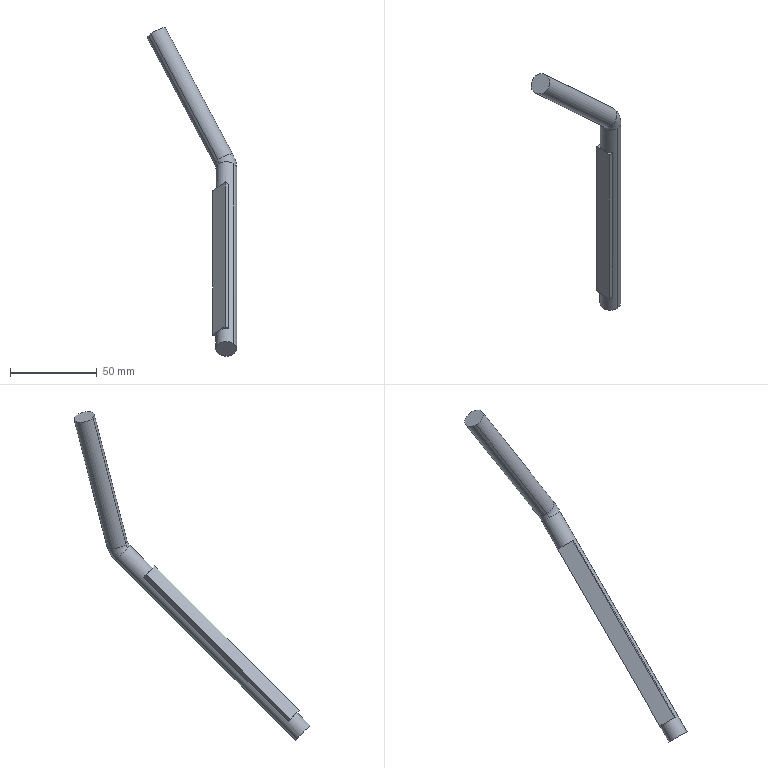Component | SolidWorks | SmallAxisAssembly-1_AdjustingRoundSteel-1 | 1 solid | 15 faces | box 51.66 x 135.82 x 189.07 mm | volume 27818 mm3 | plane 9 | cylinder 4 | torus 2 | commonest cylinder face diameters 12 x4
build123d program:
from build123d import *

# Parameters (mm, degrees)
SKETCH2_R           = 6
BOSS_EXTRUDE1_DEPTH = 6


with BuildPart() as part:
    # Sweep1: sweep along a path in Sketch1
    with BuildLine(Plane.XY) as sweep1_path:
        Line((0, 0), (146.36, 0))
        ThreePointArc((146.36, 0), (149.78, -0.6031), (152.788, -2.34))
        Line((152.788, -2.34), (217.412, -56.565))
    # Sketch2 → Sweep1 (sweep)
    with BuildSketch(Plane(origin=(0, 0, 0), x_dir=(0, 0, -1), z_dir=(1, 0, 0))):
        Circle(SKETCH2_R)
    sweep(path=sweep1_path.line)

    # Sketch3 → Boss-Extrude1 (add)
    with BuildSketch(Plane(origin=(0, -6, 0), x_dir=(1, 0, 0), z_dir=(0, 1, 0))):
        Polygon((128.068, 0), (128.068, -5), (10.576, -5), (10.576, 5), (128.068, 5), align=None)
    extrude(amount=BOSS_EXTRUDE1_DEPTH)


solid = part.part

# Placed as in the assembly
solid = solid.moved(Location((2.555, 759.132, 195.267), (-134.971, -44.465, -89.958)))
STEP:
#1=COLOUR_RGB('',0.7922,0.8196,0.9333);
#2=FILL_AREA_STYLE_COLOUR('',#1);
#3=FILL_AREA_STYLE('',(#2));
#4=SURFACE_STYLE_FILL_AREA(#3);
#5=SURFACE_SIDE_STYLE('',(#4));
#6=SURFACE_STYLE_USAGE(.BOTH.,#5);
#7=PRESENTATION_STYLE_ASSIGNMENT((#6));
#8=CARTESIAN_POINT('',(0.2691,33.842,11.881));
#9=VERTEX_POINT('',#8);
#10=CARTESIAN_POINT('',(0.2722,34.079,11.645));
#11=VERTEX_POINT('',#10);
#12=CARTESIAN_POINT('',(0.1036,33.962,11.762));
#13=DIRECTION('',(0.0005225,0.7071,0.7071));
#14=DIRECTION('',(0.7005,-0.5049,0.5044));
#15=AXIS2_PLACEMENT_3D('',#12,#13,#14);
#16=CIRCLE('',#15,0.2362);
#17=EDGE_CURVE('',#9,#11,#16,.T.);
#18=ORIENTED_EDGE('',*,*,#17,.T.);
#19=CARTESIAN_POINT('',(0.1672,34.292,12.004));
#20=VERTEX_POINT('',#19);
#21=CARTESIAN_POINT('',(-0.1774,33.767,11.957));
#22=DIRECTION('',(0.7005,-0.5049,0.5044));
#23=DIRECTION('',(0.5847,0.8112,0.));
#24=AXIS2_PLACEMENT_3D('',#21,#22,#23);
#25=CIRCLE('',#24,0.6299);
#26=EDGE_CURVE('',#11,#20,#25,.T.);
#27=ORIENTED_EDGE('',*,*,#26,.T.);
#28=CARTESIAN_POINT('',(-0.09123,33.898,11.969));
#29=VERTEX_POINT('',#28);
#30=CARTESIAN_POINT('',(0.03799,34.095,11.987));
#31=DIRECTION('',(-0.4583,0.2235,0.8602));
#32=DIRECTION('',(0.7005,-0.5049,0.5044));
#33=AXIS2_PLACEMENT_3D('',#30,#31,#32);
#34=CIRCLE('',#33,0.2362);
#35=EDGE_CURVE('',#29,#20,#34,.T.);
#36=ORIENTED_EDGE('',*,*,#35,.F.);
#37=CARTESIAN_POINT('',(-0.06499,33.845,11.879));
#38=VERTEX_POINT('',#37);
#39=CARTESIAN_POINT('',(-0.1774,33.767,11.957));
#40=DIRECTION('',(0.7005,-0.5049,0.5044));
#41=DIRECTION('',(0.5847,0.8112,0.));
#42=AXIS2_PLACEMENT_3D('',#39,#40,#41);
#43=CIRCLE('',#42,0.1575);
#44=EDGE_CURVE('',#38,#29,#43,.T.);
#45=ORIENTED_EDGE('',*,*,#44,.F.);
#46=CARTESIAN_POINT('',(0.1036,33.962,11.762));
#47=DIRECTION('',(0.0005225,0.7071,0.7071));
#48=DIRECTION('',(0.7005,-0.5049,0.5044));
#49=AXIS2_PLACEMENT_3D('',#46,#47,#48);
#50=CIRCLE('',#49,0.2362);
#51=EDGE_CURVE('',#38,#9,#50,.T.);
#52=ORIENTED_EDGE('',*,*,#51,.T.);
#53=EDGE_LOOP('',(#18,#27,#36,#45,#52));
#54=FACE_OUTER_BOUND('',#53,.T.);
#55=CARTESIAN_POINT('',(-0.1774,33.767,11.957));
#56=DIRECTION('',(0.7005,-0.5049,0.5044));
#57=DIRECTION('',(-0.0005225,-0.7071,-0.7071));
#58=AXIS2_PLACEMENT_3D('',#55,#56,#57);
#59=TOROIDAL_SURFACE('',#58,0.3937,0.2362);
#60=ADVANCED_FACE('',(#54),#59,.T.);
#61=CARTESIAN_POINT('',(0.03799,34.095,11.987));
#62=DIRECTION('',(-0.4583,0.2235,0.8602));
#63=DIRECTION('',(0.7005,-0.5049,0.5044));
#64=AXIS2_PLACEMENT_3D('',#61,#62,#63);
#65=CIRCLE('',#64,0.2362);
#66=EDGE_CURVE('',#20,#29,#65,.T.);
#67=ORIENTED_EDGE('',*,*,#66,.T.);
#68=CARTESIAN_POINT('',(-1.614,34.64,14.826));
#69=VERTEX_POINT('',#68);
#70=CARTESIAN_POINT('',(-0.09123,33.898,11.969));
#71=DIRECTION('',(-0.4583,0.2235,0.8602));
#72=VECTOR('',#71,39.37);
#73=LINE('',#70,#72);
#74=EDGE_CURVE('',#29,#69,#73,.T.);
#75=ORIENTED_EDGE('',*,*,#74,.T.);
#76=CARTESIAN_POINT('',(-1.355,35.034,14.861));
#77=VERTEX_POINT('',#76);
#78=CARTESIAN_POINT('',(-1.484,34.837,14.844));
#79=DIRECTION('',(-0.4583,0.2235,0.8602));
#80=DIRECTION('',(0.7005,-0.5049,0.5044));
#81=AXIS2_PLACEMENT_3D('',#78,#79,#80);
#82=CIRCLE('',#81,0.2362);
#83=EDGE_CURVE('',#77,#69,#82,.T.);
#84=ORIENTED_EDGE('',*,*,#83,.F.);
#85=CARTESIAN_POINT('',(0.1672,34.292,12.004));
#86=DIRECTION('',(-0.4583,0.2235,0.8602));
#87=VECTOR('',#86,39.37);
#88=LINE('',#85,#87);
#89=EDGE_CURVE('',#20,#77,#88,.T.);
#90=ORIENTED_EDGE('',*,*,#89,.F.);
#91=EDGE_LOOP('',(#67,#75,#84,#90));
#92=FACE_OUTER_BOUND('',#91,.T.);
#93=CARTESIAN_POINT('',(0.03799,34.095,11.987));
#94=DIRECTION('',(-0.4583,0.2235,0.8602));
#95=DIRECTION('',(0.547,0.8337,0.07489));
#96=AXIS2_PLACEMENT_3D('',#93,#94,#95);
#97=CYLINDRICAL_SURFACE('',#96,0.2362);
#98=ADVANCED_FACE('',(#92),#97,.T.);
#99=CARTESIAN_POINT('',(0.2661,29.768,7.807));
#100=VERTEX_POINT('',#99);
#101=CARTESIAN_POINT('',(-0.06488,30.006,7.569));
#102=VERTEX_POINT('',#101);
#103=CARTESIAN_POINT('',(0.1006,29.887,7.688));
#104=DIRECTION('',(0.0005225,0.7071,0.7071));
#105=DIRECTION('',(0.7005,-0.5049,0.5044));
#106=AXIS2_PLACEMENT_3D('',#103,#104,#105);
#107=CIRCLE('',#106,0.2362);
#108=EDGE_CURVE('',#100,#102,#107,.T.);
#109=ORIENTED_EDGE('',*,*,#108,.T.);
#110=CARTESIAN_POINT('',(-0.06187,34.081,11.643));
#111=VERTEX_POINT('',#110);
#112=CARTESIAN_POINT('',(-0.06488,30.006,7.569));
#113=DIRECTION('',(0.0005225,0.7071,0.7071));
#114=VECTOR('',#113,39.37);
#115=LINE('',#112,#114);
#116=EDGE_CURVE('',#102,#111,#115,.T.);
#117=ORIENTED_EDGE('',*,*,#116,.T.);
#118=CARTESIAN_POINT('',(0.1036,33.962,11.762));
#119=DIRECTION('',(0.0005225,0.7071,0.7071));
#120=DIRECTION('',(0.7005,-0.5049,0.5044));
#121=AXIS2_PLACEMENT_3D('',#118,#119,#120);
#122=CIRCLE('',#121,0.2362);
#123=EDGE_CURVE('',#11,#111,#122,.T.);
#124=ORIENTED_EDGE('',*,*,#123,.F.);
#125=ORIENTED_EDGE('',*,*,#17,.F.);
#126=CARTESIAN_POINT('',(0.2661,29.768,7.807));
#127=DIRECTION('',(0.0005225,0.7071,0.7071));
#128=VECTOR('',#127,39.37);
#129=LINE('',#126,#128);
#130=EDGE_CURVE('',#100,#9,#129,.T.);
#131=ORIENTED_EDGE('',*,*,#130,.F.);
#132=EDGE_LOOP('',(#109,#117,#124,#125,#131));
#133=FACE_OUTER_BOUND('',#132,.T.);
#134=CARTESIAN_POINT('',(0.1006,29.887,7.688));
#135=DIRECTION('',(0.0005225,0.7071,0.7071));
#136=DIRECTION('',(0.7005,-0.5049,0.5044));
#137=AXIS2_PLACEMENT_3D('',#134,#135,#136);
#138=CYLINDRICAL_SURFACE('',#137,0.2362);
#139=ADVANCED_FACE('',(#133),#138,.T.);
#140=ORIENTED_EDGE('',*,*,#116,.F.);
#141=CARTESIAN_POINT('',(0.1006,29.887,7.688));
#142=DIRECTION('',(0.0005225,0.7071,0.7071));
#143=DIRECTION('',(0.7005,-0.5049,0.5044));
#144=AXIS2_PLACEMENT_3D('',#141,#142,#143);
#145=CIRCLE('',#144,0.2362);
#146=EDGE_CURVE('',#102,#100,#145,.T.);
#147=ORIENTED_EDGE('',*,*,#146,.T.);
#148=ORIENTED_EDGE('',*,*,#130,.T.);
#149=ORIENTED_EDGE('',*,*,#51,.F.);
#150=CARTESIAN_POINT('',(0.1036,33.962,11.762));
#151=DIRECTION('',(0.0005225,0.7071,0.7071));
#152=DIRECTION('',(0.7005,-0.5049,0.5044));
#153=AXIS2_PLACEMENT_3D('',#150,#151,#152);
#154=CIRCLE('',#153,0.2362);
#155=EDGE_CURVE('',#111,#38,#154,.T.);
#156=ORIENTED_EDGE('',*,*,#155,.F.);
#157=EDGE_LOOP('',(#140,#147,#148,#149,#156));
#158=FACE_OUTER_BOUND('',#157,.T.);
#159=CARTESIAN_POINT('',(-0.1303,30.216,7.948));
#160=VERTEX_POINT('',#159);
#161=CARTESIAN_POINT('',(-0.1279,33.487,11.218));
#162=VERTEX_POINT('',#161);
#163=CARTESIAN_POINT('',(-0.1305,29.922,7.653));
#164=DIRECTION('',(0.0005225,0.7071,0.7071));
#165=VECTOR('',#164,39.37);
#166=LINE('',#163,#165);
#167=EDGE_CURVE('',#160,#162,#166,.T.);
#168=ORIENTED_EDGE('',*,*,#167,.T.);
#169=CARTESIAN_POINT('',(-0.06536,33.335,11.37));
#170=VERTEX_POINT('',#169);
#171=CARTESIAN_POINT('',(0.1032,33.452,11.253));
#172=DIRECTION('',(0.0005225,0.7071,0.7071));
#173=DIRECTION('',(-0.7005,0.5049,-0.5044));
#174=AXIS2_PLACEMENT_3D('',#171,#172,#173);
#175=CIRCLE('',#174,0.2362);
#176=EDGE_CURVE('',#162,#170,#175,.T.);
#177=ORIENTED_EDGE('',*,*,#176,.T.);
#178=CARTESIAN_POINT('',(0.1479,33.288,11.417));
#179=VERTEX_POINT('',#178);
#180=CARTESIAN_POINT('',(0.1032,33.452,11.253));
#181=DIRECTION('',(0.0005225,0.7071,0.7071));
#182=DIRECTION('',(-0.7005,0.5049,-0.5044));
#183=AXIS2_PLACEMENT_3D('',#180,#181,#182);
#184=CIRCLE('',#183,0.2362);
#185=EDGE_CURVE('',#170,#179,#184,.T.);
#186=ORIENTED_EDGE('',*,*,#185,.T.);
#187=CARTESIAN_POINT('',(0.1455,30.017,8.146));
#188=VERTEX_POINT('',#187);
#189=CARTESIAN_POINT('',(0.1453,29.723,7.852));
#190=DIRECTION('',(-0.0005225,-0.7071,-0.7071));
#191=VECTOR('',#190,39.37);
#192=LINE('',#189,#191);
#193=EDGE_CURVE('',#179,#188,#192,.T.);
#194=ORIENTED_EDGE('',*,*,#193,.T.);
#195=CARTESIAN_POINT('',(-0.06778,30.065,8.099));
#196=VERTEX_POINT('',#195);
#197=CARTESIAN_POINT('',(0.1008,30.182,7.982));
#198=DIRECTION('',(-0.0005225,-0.7071,-0.7071));
#199=DIRECTION('',(0.7005,-0.5049,0.5044));
#200=AXIS2_PLACEMENT_3D('',#197,#198,#199);
#201=CIRCLE('',#200,0.2362);
#202=EDGE_CURVE('',#188,#196,#201,.T.);
#203=ORIENTED_EDGE('',*,*,#202,.T.);
#204=CARTESIAN_POINT('',(0.1008,30.182,7.982));
#205=DIRECTION('',(-0.0005225,-0.7071,-0.7071));
#206=DIRECTION('',(0.7005,-0.5049,0.5044));
#207=AXIS2_PLACEMENT_3D('',#204,#205,#206);
#208=CIRCLE('',#207,0.2362);
#209=EDGE_CURVE('',#196,#160,#208,.T.);
#210=ORIENTED_EDGE('',*,*,#209,.T.);
#211=EDGE_LOOP('',(#168,#177,#186,#194,#203,#210));
#212=FACE_BOUND('',#211,.T.);
#213=CARTESIAN_POINT('',(0.1006,29.887,7.688));
#214=DIRECTION('',(0.0005225,0.7071,0.7071));
#215=DIRECTION('',(0.7005,-0.5049,0.5044));
#216=AXIS2_PLACEMENT_3D('',#213,#214,#215);
#217=CYLINDRICAL_SURFACE('',#216,0.2362);
#218=ADVANCED_FACE('',(#158,#212),#217,.T.);
#219=ORIENTED_EDGE('',*,*,#74,.F.);
#220=ORIENTED_EDGE('',*,*,#35,.T.);
#221=ORIENTED_EDGE('',*,*,#89,.T.);
#222=CARTESIAN_POINT('',(-1.484,34.837,14.844));
#223=DIRECTION('',(-0.4583,0.2235,0.8602));
#224=DIRECTION('',(0.7005,-0.5049,0.5044));
#225=AXIS2_PLACEMENT_3D('',#222,#223,#224);
#226=CIRCLE('',#225,0.2362);
#227=EDGE_CURVE('',#69,#77,#226,.T.);
#228=ORIENTED_EDGE('',*,*,#227,.F.);
#229=EDGE_LOOP('',(#219,#220,#221,#228));
#230=FACE_OUTER_BOUND('',#229,.T.);
#231=CARTESIAN_POINT('',(0.03799,34.095,11.987));
#232=DIRECTION('',(-0.4583,0.2235,0.8602));
#233=DIRECTION('',(0.547,0.8337,0.07489));
#234=AXIS2_PLACEMENT_3D('',#231,#232,#233);
#235=CYLINDRICAL_SURFACE('',#234,0.2362);
#236=ADVANCED_FACE('',(#230),#235,.T.);
#237=ORIENTED_EDGE('',*,*,#26,.F.);
#238=ORIENTED_EDGE('',*,*,#123,.T.);
#239=ORIENTED_EDGE('',*,*,#155,.T.);
#240=ORIENTED_EDGE('',*,*,#44,.T.);
#241=ORIENTED_EDGE('',*,*,#66,.F.);
#242=EDGE_LOOP('',(#237,#238,#239,#240,#241));
#243=FACE_OUTER_BOUND('',#242,.T.);
#244=CARTESIAN_POINT('',(-0.1774,33.767,11.957));
#245=DIRECTION('',(0.7005,-0.5049,0.5044));
#246=DIRECTION('',(-0.0005225,-0.7071,-0.7071));
#247=AXIS2_PLACEMENT_3D('',#244,#245,#246);
#248=TOROIDAL_SURFACE('',#247,0.3937,0.2362);
#249=ADVANCED_FACE('',(#243),#248,.T.);
#250=ORIENTED_EDGE('',*,*,#83,.T.);
#251=ORIENTED_EDGE('',*,*,#227,.T.);
#252=EDGE_LOOP('',(#250,#251));
#253=FACE_OUTER_BOUND('',#252,.T.);
#254=CARTESIAN_POINT('',(-1.484,34.837,14.844));
#255=DIRECTION('',(-0.4583,0.2235,0.8602));
#256=DIRECTION('',(0.7005,-0.5049,0.5044));
#257=AXIS2_PLACEMENT_3D('',#254,#255,#256);
#258=PLANE('',#257);
#259=ADVANCED_FACE('',(#253),#258,.T.);
#260=ORIENTED_EDGE('',*,*,#108,.F.);
#261=ORIENTED_EDGE('',*,*,#146,.F.);
#262=EDGE_LOOP('',(#260,#261));
#263=FACE_OUTER_BOUND('',#262,.T.);
#264=CARTESIAN_POINT('',(0.1006,29.887,7.688));
#265=DIRECTION('',(0.0005225,0.7071,0.7071));
#266=DIRECTION('',(0.7005,-0.5049,0.5044));
#267=AXIS2_PLACEMENT_3D('',#264,#265,#266);
#268=PLANE('',#267);
#269=ADVANCED_FACE('',(#263),#268,.F.);
#270=ORIENTED_EDGE('',*,*,#202,.F.);
#271=CARTESIAN_POINT('',(0.07011,29.965,8.198));
#272=VERTEX_POINT('',#271);
#273=CARTESIAN_POINT('',(0.2387,30.082,8.081));
#274=DIRECTION('',(-0.7137,-0.495,0.4956));
#275=VECTOR('',#274,39.37);
#276=LINE('',#273,#275);
#277=EDGE_CURVE('',#188,#272,#276,.T.);
#278=ORIENTED_EDGE('',*,*,#277,.T.);
#279=CARTESIAN_POINT('',(-0.2057,30.164,8.));
#280=DIRECTION('',(-0.7005,0.5049,-0.5044));
#281=VECTOR('',#280,39.37);
#282=LINE('',#279,#281);
#283=EDGE_CURVE('',#272,#196,#282,.T.);
#284=ORIENTED_EDGE('',*,*,#283,.T.);
#285=EDGE_LOOP('',(#270,#278,#284));
#286=FACE_OUTER_BOUND('',#285,.T.);
#287=CARTESIAN_POINT('',(-0.03708,30.281,7.883));
#288=DIRECTION('',(0.0005225,0.7071,0.7071));
#289=DIRECTION('',(0.7005,-0.5049,0.5044));
#290=AXIS2_PLACEMENT_3D('',#287,#288,#289);
#291=PLANE('',#290);
#292=ADVANCED_FACE('',(#286),#291,.F.);
#293=ORIENTED_EDGE('',*,*,#176,.F.);
#294=CARTESIAN_POINT('',(-0.2033,33.435,11.271));
#295=VERTEX_POINT('',#294);
#296=CARTESIAN_POINT('',(-0.03467,33.552,11.154));
#297=DIRECTION('',(-0.7137,-0.495,0.4956));
#298=VECTOR('',#297,39.37);
#299=LINE('',#296,#298);
#300=EDGE_CURVE('',#162,#295,#299,.T.);
#301=ORIENTED_EDGE('',*,*,#300,.T.);
#302=CARTESIAN_POINT('',(-0.06536,33.335,11.37));
#303=DIRECTION('',(0.7005,-0.5049,0.5044));
#304=VECTOR('',#303,39.37);
#305=LINE('',#302,#304);
#306=EDGE_CURVE('',#295,#170,#305,.T.);
#307=ORIENTED_EDGE('',*,*,#306,.T.);
#308=EDGE_LOOP('',(#293,#301,#307));
#309=FACE_OUTER_BOUND('',#308,.T.);
#310=CARTESIAN_POINT('',(0.1032,33.452,11.253));
#311=DIRECTION('',(-0.0005225,-0.7071,-0.7071));
#312=DIRECTION('',(-0.7005,0.5049,-0.5044));
#313=AXIS2_PLACEMENT_3D('',#310,#311,#312);
#314=PLANE('',#313);
#315=ADVANCED_FACE('',(#309),#314,.F.);
#316=CARTESIAN_POINT('',(-0.2057,30.164,8.));
#317=VERTEX_POINT('',#316);
#318=CARTESIAN_POINT('',(-0.2057,30.164,8.));
#319=DIRECTION('',(-0.7005,0.5049,-0.5044));
#320=VECTOR('',#319,39.37);
#321=LINE('',#318,#320);
#322=EDGE_CURVE('',#196,#317,#321,.T.);
#323=ORIENTED_EDGE('',*,*,#322,.F.);
#324=ORIENTED_EDGE('',*,*,#283,.F.);
#325=CARTESIAN_POINT('',(0.07253,33.236,11.469));
#326=VERTEX_POINT('',#325);
#327=CARTESIAN_POINT('',(0.07011,29.965,8.198));
#328=DIRECTION('',(-0.0005225,-0.7071,-0.7071));
#329=VECTOR('',#328,39.37);
#330=LINE('',#327,#329);
#331=EDGE_CURVE('',#326,#272,#330,.T.);
#332=ORIENTED_EDGE('',*,*,#331,.F.);
#333=CARTESIAN_POINT('',(-0.06536,33.335,11.37));
#334=DIRECTION('',(0.7005,-0.5049,0.5044));
#335=VECTOR('',#334,39.37);
#336=LINE('',#333,#335);
#337=EDGE_CURVE('',#170,#326,#336,.T.);
#338=ORIENTED_EDGE('',*,*,#337,.F.);
#339=ORIENTED_EDGE('',*,*,#306,.F.);
#340=CARTESIAN_POINT('',(-0.2033,33.435,11.271));
#341=DIRECTION('',(0.0005225,0.7071,0.7071));
#342=VECTOR('',#341,39.37);
#343=LINE('',#340,#342);
#344=EDGE_CURVE('',#317,#295,#343,.T.);
#345=ORIENTED_EDGE('',*,*,#344,.F.);
#346=EDGE_LOOP('',(#323,#324,#332,#338,#339,#345));
#347=FACE_OUTER_BOUND('',#346,.T.);
#348=CARTESIAN_POINT('',(-0.068,29.77,7.805));
#349=DIRECTION('',(-0.7137,-0.495,0.4956));
#350=DIRECTION('',(0.7005,-0.5049,0.5044));
#351=AXIS2_PLACEMENT_3D('',#348,#349,#350);
#352=PLANE('',#351);
#353=ADVANCED_FACE('',(#347),#352,.T.);
#354=ORIENTED_EDGE('',*,*,#193,.F.);
#355=CARTESIAN_POINT('',(0.2411,33.353,11.352));
#356=DIRECTION('',(-0.7137,-0.495,0.4956));
#357=VECTOR('',#356,39.37);
#358=LINE('',#355,#357);
#359=EDGE_CURVE('',#179,#326,#358,.T.);
#360=ORIENTED_EDGE('',*,*,#359,.T.);
#361=ORIENTED_EDGE('',*,*,#331,.T.);
#362=ORIENTED_EDGE('',*,*,#277,.F.);
#363=EDGE_LOOP('',(#354,#360,#361,#362));
#364=FACE_OUTER_BOUND('',#363,.T.);
#365=CARTESIAN_POINT('',(0.2387,30.082,8.081));
#366=DIRECTION('',(-0.7005,0.5049,-0.5044));
#367=DIRECTION('',(0.0005225,0.7071,0.7071));
#368=AXIS2_PLACEMENT_3D('',#365,#366,#367);
#369=PLANE('',#368);
#370=ADVANCED_FACE('',(#364),#369,.F.);
#371=ORIENTED_EDGE('',*,*,#209,.F.);
#372=ORIENTED_EDGE('',*,*,#322,.T.);
#373=CARTESIAN_POINT('',(-0.03708,30.281,7.883));
#374=DIRECTION('',(-0.7137,-0.495,0.4956));
#375=VECTOR('',#374,39.37);
#376=LINE('',#373,#375);
#377=EDGE_CURVE('',#160,#317,#376,.T.);
#378=ORIENTED_EDGE('',*,*,#377,.F.);
#379=EDGE_LOOP('',(#371,#372,#378));
#380=FACE_OUTER_BOUND('',#379,.T.);
#381=CARTESIAN_POINT('',(-0.03708,30.281,7.883));
#382=DIRECTION('',(0.0005225,0.7071,0.7071));
#383=DIRECTION('',(0.7005,-0.5049,0.5044));
#384=AXIS2_PLACEMENT_3D('',#381,#382,#383);
#385=PLANE('',#384);
#386=ADVANCED_FACE('',(#380),#385,.F.);
#387=ORIENTED_EDGE('',*,*,#167,.F.);
#388=ORIENTED_EDGE('',*,*,#377,.T.);
#389=ORIENTED_EDGE('',*,*,#344,.T.);
#390=ORIENTED_EDGE('',*,*,#300,.F.);
#391=EDGE_LOOP('',(#387,#388,#389,#390));
#392=FACE_OUTER_BOUND('',#391,.T.);
#393=CARTESIAN_POINT('',(-0.03467,33.552,11.154));
#394=DIRECTION('',(0.7005,-0.5049,0.5044));
#395=DIRECTION('',(-0.0005225,-0.7071,-0.7071));
#396=AXIS2_PLACEMENT_3D('',#393,#394,#395);
#397=PLANE('',#396);
#398=ADVANCED_FACE('',(#392),#397,.F.);
#399=ORIENTED_EDGE('',*,*,#185,.F.);
#400=ORIENTED_EDGE('',*,*,#337,.T.);
#401=ORIENTED_EDGE('',*,*,#359,.F.);
#402=EDGE_LOOP('',(#399,#400,#401));
#403=FACE_OUTER_BOUND('',#402,.T.);
#404=CARTESIAN_POINT('',(0.1032,33.452,11.253));
#405=DIRECTION('',(-0.0005225,-0.7071,-0.7071));
#406=DIRECTION('',(-0.7005,0.5049,-0.5044));
#407=AXIS2_PLACEMENT_3D('',#404,#405,#406);
#408=PLANE('',#407);
#409=ADVANCED_FACE('',(#403),#408,.F.);
#410=CLOSED_SHELL('',(#60,#98,#139,#218,#236,#249,#259,#269,#292,#315,#353,#370,#386,#398,#409));
#411=MANIFOLD_SOLID_BREP('',#410);
#412=STYLED_ITEM('',(#7),#411);
#413=(LENGTH_UNIT()NAMED_UNIT(*)SI_UNIT($,.METRE.));
#414=LENGTH_MEASURE_WITH_UNIT(LENGTH_MEASURE(0.0254),#413);
#415=DIMENSIONAL_EXPONENTS(1.,0.,0.,0.,0.,0.,0.);
#416=(CONVERSION_BASED_UNIT('',#414)LENGTH_UNIT()NAMED_UNIT(#415));
#417=UNCERTAINTY_MEASURE_WITH_UNIT(LENGTH_MEASURE(0.00001),#416,'','');
#418=(NAMED_UNIT(*)PLANE_ANGLE_UNIT()SI_UNIT($,.RADIAN.));
#419=(NAMED_UNIT(*)SI_UNIT($,.STERADIAN.)SOLID_ANGLE_UNIT());
#420=(GEOMETRIC_REPRESENTATION_CONTEXT(3)GLOBAL_UNCERTAINTY_ASSIGNED_CONTEXT((#417))GLOBAL_UNIT_ASSIGNED_CONTEXT((#416,#418,#419))REPRESENTATION_CONTEXT('',''));
#421=MECHANICAL_DESIGN_GEOMETRIC_PRESENTATION_REPRESENTATION('',(#412),#420);
#422=PRESENTATION_LAYER_ASSIGNMENT('','',(#412));
#423=CARTESIAN_POINT('',(0.,0.,0.));
#424=DIRECTION('',(0.,0.,1.));
#425=DIRECTION('',(1.,0.,0.));
#426=AXIS2_PLACEMENT_3D('',#423,#424,#425);
#427=(LENGTH_UNIT()NAMED_UNIT(*)SI_UNIT($,.METRE.));
#428=LENGTH_MEASURE_WITH_UNIT(LENGTH_MEASURE(0.0254),#427);
#429=DIMENSIONAL_EXPONENTS(1.,0.,0.,0.,0.,0.,0.);
#430=(CONVERSION_BASED_UNIT('',#428)LENGTH_UNIT()NAMED_UNIT(#429));
#431=UNCERTAINTY_MEASURE_WITH_UNIT(LENGTH_MEASURE(0.00001),#430,'','');
#432=(NAMED_UNIT(*)PLANE_ANGLE_UNIT()SI_UNIT($,.RADIAN.));
#433=(NAMED_UNIT(*)SI_UNIT($,.STERADIAN.)SOLID_ANGLE_UNIT());
#434=(GEOMETRIC_REPRESENTATION_CONTEXT(3)GLOBAL_UNCERTAINTY_ASSIGNED_CONTEXT((#431))GLOBAL_UNIT_ASSIGNED_CONTEXT((#430,#432,#433))REPRESENTATION_CONTEXT('',''));
#435=ADVANCED_BREP_SHAPE_REPRESENTATION('',(#411,#426),#434);